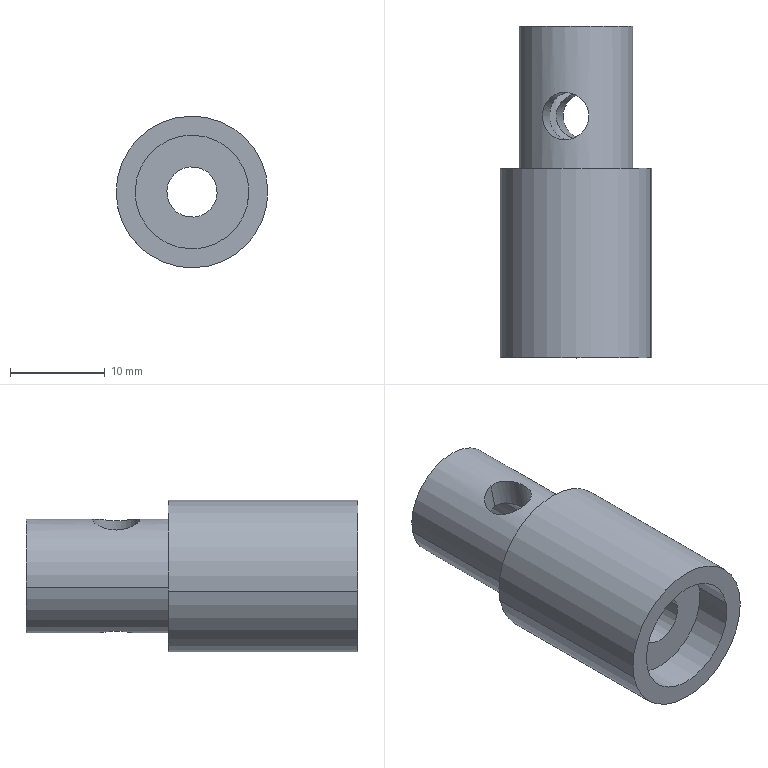Component | SolidWorks | UltrasonicProductSuction-10_SuctionPositioning-1 | 1 solid | 19 faces | box 16 x 35 x 16 mm | volume 4290 mm3 | cylinder 14 | plane 5 | commonest cylinder face diameters 5 x4 12 x4 5.3 x2 16 x2 6 x2 | material AISI 304
STEP:
#1=COLOUR_RGB('',0.7922,0.8196,0.9333);
#2=FILL_AREA_STYLE_COLOUR('',#1);
#3=FILL_AREA_STYLE('',(#2));
#4=SURFACE_STYLE_FILL_AREA(#3);
#5=SURFACE_SIDE_STYLE('',(#4));
#6=SURFACE_STYLE_USAGE(.BOTH.,#5);
#7=PRESENTATION_STYLE_ASSIGNMENT((#6));
#8=CARTESIAN_POINT('',(68.99,150.659,43.813));
#9=VERTEX_POINT('',#8);
#10=CARTESIAN_POINT('',(68.99,150.855,43.813));
#11=VERTEX_POINT('',#10);
#12=CARTESIAN_POINT('',(68.99,150.659,43.813));
#13=CARTESIAN_POINT('',(68.984,150.659,43.812));
#14=CARTESIAN_POINT('',(68.978,150.659,43.811));
#15=CARTESIAN_POINT('',(68.965,150.662,43.81));
#16=CARTESIAN_POINT('',(68.959,150.664,43.809));
#17=CARTESIAN_POINT('',(68.941,150.671,43.808));
#18=CARTESIAN_POINT('',(68.929,150.678,43.809));
#19=CARTESIAN_POINT('',(68.915,150.692,43.81));
#20=CARTESIAN_POINT('',(68.911,150.697,43.811));
#21=CARTESIAN_POINT('',(68.904,150.708,43.812));
#22=CARTESIAN_POINT('',(68.9,150.713,43.813));
#23=CARTESIAN_POINT('',(68.895,150.725,43.814));
#24=CARTESIAN_POINT('',(68.893,150.731,43.814));
#25=CARTESIAN_POINT('',(68.89,150.744,43.815));
#26=CARTESIAN_POINT('',(68.89,150.75,43.815));
#27=CARTESIAN_POINT('',(68.89,150.77,43.815));
#28=CARTESIAN_POINT('',(68.892,150.783,43.814));
#29=CARTESIAN_POINT('',(68.9,150.801,43.813));
#30=CARTESIAN_POINT('',(68.904,150.807,43.812));
#31=CARTESIAN_POINT('',(68.911,150.817,43.811));
#32=CARTESIAN_POINT('',(68.915,150.822,43.81));
#33=CARTESIAN_POINT('',(68.929,150.836,43.809));
#34=CARTESIAN_POINT('',(68.941,150.843,43.808));
#35=CARTESIAN_POINT('',(68.959,150.85,43.809));
#36=CARTESIAN_POINT('',(68.965,150.852,43.81));
#37=CARTESIAN_POINT('',(68.978,150.855,43.811));
#38=CARTESIAN_POINT('',(68.984,150.855,43.812));
#39=CARTESIAN_POINT('',(68.99,150.855,43.813));
#40=B_SPLINE_CURVE_WITH_KNOTS('',3,(#12,#13,#14,#15,#16,#17,#18,#19,#20,#21,#22,#23,#24,#25,#26,#27,#28,#29,#30,#31,#32,#33,#34,#35,#36,#37,#38,#39),.UNSPECIFIED.,.F.,.F.,(4,2,2,2,2,2,2,2,2,2,2,2,2,4),(0.00756,0.008054,0.008548,0.009536,0.01003,0.01052,0.01102,0.01151,0.0125,0.01299,0.01349,0.01447,0.01497,0.01546),.UNSPECIFIED.);
#41=EDGE_CURVE('',#9,#11,#40,.T.);
#42=ORIENTED_EDGE('',*,*,#41,.T.);
#43=CARTESIAN_POINT('',(68.967,150.855,43.929));
#44=VERTEX_POINT('',#43);
#45=CARTESIAN_POINT('',(69.006,150.855,43.736));
#46=DIRECTION('',(-0.1987,-0.00003085,0.9801));
#47=VECTOR('',#46,39.37);
#48=LINE('',#45,#47);
#49=EDGE_CURVE('',#11,#44,#48,.T.);
#50=ORIENTED_EDGE('',*,*,#49,.T.);
#51=CARTESIAN_POINT('',(68.967,150.659,43.929));
#52=VERTEX_POINT('',#51);
#53=CARTESIAN_POINT('',(68.967,150.659,43.929));
#54=CARTESIAN_POINT('',(68.96,150.659,43.928));
#55=CARTESIAN_POINT('',(68.953,150.659,43.927));
#56=CARTESIAN_POINT('',(68.94,150.662,43.927));
#57=CARTESIAN_POINT('',(68.933,150.664,43.927));
#58=CARTESIAN_POINT('',(68.921,150.669,43.929));
#59=CARTESIAN_POINT('',(68.915,150.673,43.93));
#60=CARTESIAN_POINT('',(68.903,150.68,43.934));
#61=CARTESIAN_POINT('',(68.898,150.684,43.936));
#62=CARTESIAN_POINT('',(68.889,150.693,43.94));
#63=CARTESIAN_POINT('',(68.884,150.697,43.943));
#64=CARTESIAN_POINT('',(68.876,150.707,43.948));
#65=CARTESIAN_POINT('',(68.873,150.713,43.95));
#66=CARTESIAN_POINT('',(68.867,150.724,43.955));
#67=CARTESIAN_POINT('',(68.864,150.73,43.957));
#68=CARTESIAN_POINT('',(68.862,150.74,43.96));
#69=CARTESIAN_POINT('',(68.861,150.743,43.96));
#70=CARTESIAN_POINT('',(68.86,150.75,43.961));
#71=CARTESIAN_POINT('',(68.86,150.754,43.961));
#72=CARTESIAN_POINT('',(68.86,150.764,43.961));
#73=CARTESIAN_POINT('',(68.861,150.771,43.96));
#74=CARTESIAN_POINT('',(68.864,150.784,43.957));
#75=CARTESIAN_POINT('',(68.867,150.79,43.955));
#76=CARTESIAN_POINT('',(68.873,150.801,43.95));
#77=CARTESIAN_POINT('',(68.876,150.807,43.948));
#78=CARTESIAN_POINT('',(68.884,150.817,43.943));
#79=CARTESIAN_POINT('',(68.889,150.821,43.94));
#80=CARTESIAN_POINT('',(68.898,150.83,43.936));
#81=CARTESIAN_POINT('',(68.903,150.834,43.934));
#82=CARTESIAN_POINT('',(68.915,150.841,43.93));
#83=CARTESIAN_POINT('',(68.92,150.844,43.929));
#84=CARTESIAN_POINT('',(68.933,150.85,43.927));
#85=CARTESIAN_POINT('',(68.94,150.852,43.927));
#86=CARTESIAN_POINT('',(68.953,150.855,43.927));
#87=CARTESIAN_POINT('',(68.96,150.855,43.928));
#88=CARTESIAN_POINT('',(68.967,150.855,43.929));
#89=B_SPLINE_CURVE_WITH_KNOTS('',3,(#53,#54,#55,#56,#57,#58,#59,#60,#61,#62,#63,#64,#65,#66,#67,#68,#69,#70,#71,#72,#73,#74,#75,#76,#77,#78,#79,#80,#81,#82,#83,#84,#85,#86,#87,#88),.UNSPECIFIED.,.F.,.F.,(4,2,2,2,2,2,2,2,2,2,2,2,2,2,2,2,2,4),(0.008234,0.008754,0.009273,0.009792,0.01031,0.01083,0.01135,0.01187,0.01213,0.01239,0.01291,0.01343,0.01395,0.01447,0.01499,0.01551,0.01602,0.01654),.UNSPECIFIED.);
#90=EDGE_CURVE('',#52,#44,#89,.T.);
#91=ORIENTED_EDGE('',*,*,#90,.F.);
#92=CARTESIAN_POINT('',(69.006,150.659,43.736));
#93=DIRECTION('',(-0.1987,-0.00003085,0.9801));
#94=VECTOR('',#93,39.37);
#95=LINE('',#92,#94);
#96=EDGE_CURVE('',#9,#52,#95,.T.);
#97=ORIENTED_EDGE('',*,*,#96,.F.);
#98=EDGE_LOOP('',(#42,#50,#91,#97));
#99=FACE_OUTER_BOUND('',#98,.T.);
#100=CARTESIAN_POINT('',(69.006,150.757,43.736));
#101=DIRECTION('',(-0.1987,-0.00003085,0.9801));
#102=DIRECTION('',(0.0001552,-1.,0.));
#103=AXIS2_PLACEMENT_3D('',#100,#101,#102);
#104=CYLINDRICAL_SURFACE('',#103,0.09843);
#105=ADVANCED_FACE('',(#99),#104,.F.);
#106=CARTESIAN_POINT('',(68.92,150.855,44.161));
#107=VERTEX_POINT('',#106);
#108=CARTESIAN_POINT('',(68.92,150.659,44.161));
#109=VERTEX_POINT('',#108);
#110=CARTESIAN_POINT('',(68.92,150.855,44.161));
#111=CARTESIAN_POINT('',(68.913,150.855,44.159));
#112=CARTESIAN_POINT('',(68.907,150.855,44.157));
#113=CARTESIAN_POINT('',(68.894,150.852,44.152));
#114=CARTESIAN_POINT('',(68.888,150.85,44.149));
#115=CARTESIAN_POINT('',(68.872,150.842,44.14));
#116=CARTESIAN_POINT('',(68.863,150.835,44.132));
#117=CARTESIAN_POINT('',(68.849,150.817,44.116));
#118=CARTESIAN_POINT('',(68.843,150.807,44.108));
#119=CARTESIAN_POINT('',(68.838,150.79,44.098));
#120=CARTESIAN_POINT('',(68.836,150.784,44.095));
#121=CARTESIAN_POINT('',(68.835,150.774,44.092));
#122=CARTESIAN_POINT('',(68.835,150.771,44.091));
#123=CARTESIAN_POINT('',(68.834,150.764,44.09));
#124=CARTESIAN_POINT('',(68.834,150.761,44.089));
#125=CARTESIAN_POINT('',(68.834,150.75,44.089));
#126=CARTESIAN_POINT('',(68.835,150.743,44.091));
#127=CARTESIAN_POINT('',(68.836,150.73,44.095));
#128=CARTESIAN_POINT('',(68.838,150.724,44.098));
#129=CARTESIAN_POINT('',(68.843,150.707,44.108));
#130=CARTESIAN_POINT('',(68.848,150.697,44.116));
#131=CARTESIAN_POINT('',(68.863,150.679,44.132));
#132=CARTESIAN_POINT('',(68.872,150.672,44.14));
#133=CARTESIAN_POINT('',(68.888,150.664,44.149));
#134=CARTESIAN_POINT('',(68.894,150.662,44.152));
#135=CARTESIAN_POINT('',(68.907,150.659,44.157));
#136=CARTESIAN_POINT('',(68.913,150.659,44.159));
#137=CARTESIAN_POINT('',(68.92,150.659,44.161));
#138=B_SPLINE_CURVE_WITH_KNOTS('',3,(#110,#111,#112,#113,#114,#115,#116,#117,#118,#119,#120,#121,#122,#123,#124,#125,#126,#127,#128,#129,#130,#131,#132,#133,#134,#135,#136,#137),.UNSPECIFIED.,.F.,.F.,(4,2,2,2,2,2,2,2,2,2,2,2,2,4),(0.01654,0.01707,0.01759,0.01863,0.01967,0.02019,0.02045,0.02071,0.02123,0.02175,0.0228,0.02384,0.02436,0.02488),.UNSPECIFIED.);
#139=EDGE_CURVE('',#107,#109,#138,.T.);
#140=ORIENTED_EDGE('',*,*,#139,.F.);
#141=CARTESIAN_POINT('',(68.897,150.855,44.276));
#142=VERTEX_POINT('',#141);
#143=CARTESIAN_POINT('',(69.006,150.855,43.736));
#144=DIRECTION('',(-0.1987,-0.00003085,0.9801));
#145=VECTOR('',#144,39.37);
#146=LINE('',#143,#145);
#147=EDGE_CURVE('',#107,#142,#146,.T.);
#148=ORIENTED_EDGE('',*,*,#147,.T.);
#149=CARTESIAN_POINT('',(68.897,150.659,44.276));
#150=VERTEX_POINT('',#149);
#151=CARTESIAN_POINT('',(68.897,150.855,44.276));
#152=CARTESIAN_POINT('',(68.89,150.855,44.275));
#153=CARTESIAN_POINT('',(68.884,150.855,44.274));
#154=CARTESIAN_POINT('',(68.871,150.852,44.27));
#155=CARTESIAN_POINT('',(68.866,150.85,44.268));
#156=CARTESIAN_POINT('',(68.854,150.845,44.264));
#157=CARTESIAN_POINT('',(68.849,150.842,44.261));
#158=CARTESIAN_POINT('',(68.839,150.835,44.257));
#159=CARTESIAN_POINT('',(68.834,150.831,44.255));
#160=CARTESIAN_POINT('',(68.826,150.822,44.25));
#161=CARTESIAN_POINT('',(68.822,150.817,44.248));
#162=CARTESIAN_POINT('',(68.816,150.806,44.244));
#163=CARTESIAN_POINT('',(68.813,150.801,44.242));
#164=CARTESIAN_POINT('',(68.809,150.789,44.239));
#165=CARTESIAN_POINT('',(68.807,150.783,44.238));
#166=CARTESIAN_POINT('',(68.805,150.77,44.236));
#167=CARTESIAN_POINT('',(68.804,150.763,44.236));
#168=CARTESIAN_POINT('',(68.804,150.75,44.236));
#169=CARTESIAN_POINT('',(68.805,150.744,44.236));
#170=CARTESIAN_POINT('',(68.807,150.731,44.238));
#171=CARTESIAN_POINT('',(68.809,150.725,44.239));
#172=CARTESIAN_POINT('',(68.813,150.713,44.242));
#173=CARTESIAN_POINT('',(68.816,150.707,44.244));
#174=CARTESIAN_POINT('',(68.823,150.697,44.248));
#175=CARTESIAN_POINT('',(68.826,150.692,44.25));
#176=CARTESIAN_POINT('',(68.835,150.683,44.255));
#177=CARTESIAN_POINT('',(68.839,150.679,44.257));
#178=CARTESIAN_POINT('',(68.849,150.672,44.262));
#179=CARTESIAN_POINT('',(68.854,150.669,44.264));
#180=CARTESIAN_POINT('',(68.871,150.661,44.27));
#181=CARTESIAN_POINT('',(68.884,150.659,44.274));
#182=CARTESIAN_POINT('',(68.897,150.659,44.276));
#183=B_SPLINE_CURVE_WITH_KNOTS('',3,(#151,#152,#153,#154,#155,#156,#157,#158,#159,#160,#161,#162,#163,#164,#165,#166,#167,#168,#169,#170,#171,#172,#173,#174,#175,#176,#177,#178,#179,#180,#181,#182),.UNSPECIFIED.,.F.,.F.,(4,2,2,2,2,2,2,2,2,2,2,2,2,2,2,4),(0.01546,0.01596,0.01645,0.01694,0.01744,0.01793,0.01843,0.01892,0.01941,0.01991,0.0204,0.0209,0.02139,0.02188,0.02238,0.02337),.UNSPECIFIED.);
#184=EDGE_CURVE('',#142,#150,#183,.T.);
#185=ORIENTED_EDGE('',*,*,#184,.T.);
#186=CARTESIAN_POINT('',(69.006,150.659,43.736));
#187=DIRECTION('',(-0.1987,-0.00003085,0.9801));
#188=VECTOR('',#187,39.37);
#189=LINE('',#186,#188);
#190=EDGE_CURVE('',#109,#150,#189,.T.);
#191=ORIENTED_EDGE('',*,*,#190,.F.);
#192=EDGE_LOOP('',(#140,#148,#185,#191));
#193=FACE_OUTER_BOUND('',#192,.T.);
#194=CARTESIAN_POINT('',(69.006,150.757,43.736));
#195=DIRECTION('',(-0.1987,-0.00003085,0.9801));
#196=DIRECTION('',(0.0001552,-1.,0.));
#197=AXIS2_PLACEMENT_3D('',#194,#195,#196);
#198=CYLINDRICAL_SURFACE('',#197,0.09843);
#199=ADVANCED_FACE('',(#193),#198,.F.);
#200=CARTESIAN_POINT('',(68.841,149.911,44.024));
#201=VERTEX_POINT('',#200);
#202=CARTESIAN_POINT('',(69.046,149.911,44.066));
#203=VERTEX_POINT('',#202);
#204=CARTESIAN_POINT('',(68.944,149.911,44.045));
#205=DIRECTION('',(0.0001552,-1.,0.));
#206=DIRECTION('',(0.9801,0.0001522,0.1987));
#207=AXIS2_PLACEMENT_3D('',#204,#205,#206);
#208=CIRCLE('',#207,0.1043);
#209=EDGE_CURVE('',#201,#203,#208,.T.);
#210=ORIENTED_EDGE('',*,*,#209,.T.);
#211=CARTESIAN_POINT('',(69.046,150.068,44.066));
#212=VERTEX_POINT('',#211);
#213=CARTESIAN_POINT('',(69.046,149.871,44.066));
#214=DIRECTION('',(-0.0001552,1.,-0.));
#215=VECTOR('',#214,39.37);
#216=LINE('',#213,#215);
#217=EDGE_CURVE('',#203,#212,#216,.T.);
#218=ORIENTED_EDGE('',*,*,#217,.T.);
#219=CARTESIAN_POINT('',(68.841,150.068,44.024));
#220=VERTEX_POINT('',#219);
#221=CARTESIAN_POINT('',(68.944,150.068,44.045));
#222=DIRECTION('',(-0.0001552,1.,-0.));
#223=DIRECTION('',(-0.9801,-0.0001522,-0.1987));
#224=AXIS2_PLACEMENT_3D('',#221,#222,#223);
#225=CIRCLE('',#224,0.1043);
#226=EDGE_CURVE('',#212,#220,#225,.T.);
#227=ORIENTED_EDGE('',*,*,#226,.T.);
#228=CARTESIAN_POINT('',(68.841,149.871,44.024));
#229=DIRECTION('',(-0.0001552,1.,-0.));
#230=VECTOR('',#229,39.37);
#231=LINE('',#228,#230);
#232=EDGE_CURVE('',#201,#220,#231,.T.);
#233=ORIENTED_EDGE('',*,*,#232,.F.);
#234=EDGE_LOOP('',(#210,#218,#227,#233));
#235=FACE_OUTER_BOUND('',#234,.T.);
#236=CARTESIAN_POINT('',(68.944,149.871,44.045));
#237=DIRECTION('',(-0.0001552,1.,-0.));
#238=DIRECTION('',(-0.9801,-0.0001522,-0.1987));
#239=AXIS2_PLACEMENT_3D('',#236,#237,#238);
#240=CYLINDRICAL_SURFACE('',#239,0.1043);
#241=ADVANCED_FACE('',(#235),#240,.F.);
#242=CARTESIAN_POINT('',(68.712,149.911,43.998));
#243=VERTEX_POINT('',#242);
#244=CARTESIAN_POINT('',(69.175,149.911,44.092));
#245=VERTEX_POINT('',#244);
#246=CARTESIAN_POINT('',(68.944,149.911,44.045));
#247=DIRECTION('',(0.0001552,-1.,0.));
#248=DIRECTION('',(0.9801,0.0001522,0.1987));
#249=AXIS2_PLACEMENT_3D('',#246,#247,#248);
#250=CIRCLE('',#249,0.2362);
#251=EDGE_CURVE('',#243,#245,#250,.T.);
#252=ORIENTED_EDGE('',*,*,#251,.F.);
#253=CARTESIAN_POINT('',(68.712,149.753,43.998));
#254=VERTEX_POINT('',#253);
#255=CARTESIAN_POINT('',(68.712,149.911,43.998));
#256=DIRECTION('',(0.0001552,-1.,0.));
#257=VECTOR('',#256,39.37);
#258=LINE('',#255,#257);
#259=EDGE_CURVE('',#243,#254,#258,.T.);
#260=ORIENTED_EDGE('',*,*,#259,.T.);
#261=CARTESIAN_POINT('',(69.175,149.753,44.092));
#262=VERTEX_POINT('',#261);
#263=CARTESIAN_POINT('',(68.944,149.753,44.045));
#264=DIRECTION('',(0.0001552,-1.,0.));
#265=DIRECTION('',(0.9801,0.0001522,0.1987));
#266=AXIS2_PLACEMENT_3D('',#263,#264,#265);
#267=CIRCLE('',#266,0.2362);
#268=EDGE_CURVE('',#254,#262,#267,.T.);
#269=ORIENTED_EDGE('',*,*,#268,.T.);
#270=CARTESIAN_POINT('',(69.175,149.911,44.092));
#271=DIRECTION('',(0.0001552,-1.,0.));
#272=VECTOR('',#271,39.37);
#273=LINE('',#270,#272);
#274=EDGE_CURVE('',#245,#262,#273,.T.);
#275=ORIENTED_EDGE('',*,*,#274,.F.);
#276=EDGE_LOOP('',(#252,#260,#269,#275));
#277=FACE_OUTER_BOUND('',#276,.T.);
#278=CARTESIAN_POINT('',(68.944,149.911,44.045));
#279=DIRECTION('',(0.0001552,-1.,0.));
#280=DIRECTION('',(0.9801,0.0001522,0.1987));
#281=AXIS2_PLACEMENT_3D('',#278,#279,#280);
#282=CYLINDRICAL_SURFACE('',#281,0.2362);
#283=ADVANCED_FACE('',(#277),#282,.F.);
#284=CARTESIAN_POINT('',(69.252,149.753,44.108));
#285=VERTEX_POINT('',#284);
#286=CARTESIAN_POINT('',(68.635,149.753,43.982));
#287=VERTEX_POINT('',#286);
#288=CARTESIAN_POINT('',(68.944,149.753,44.045));
#289=DIRECTION('',(0.0001552,-1.,0.));
#290=DIRECTION('',(0.9801,0.0001522,0.1987));
#291=AXIS2_PLACEMENT_3D('',#288,#289,#290);
#292=CIRCLE('',#291,0.315);
#293=EDGE_CURVE('',#285,#287,#292,.T.);
#294=ORIENTED_EDGE('',*,*,#293,.F.);
#295=CARTESIAN_POINT('',(69.252,150.541,44.108));
#296=VERTEX_POINT('',#295);
#297=CARTESIAN_POINT('',(69.252,149.556,44.108));
#298=DIRECTION('',(-0.0001552,1.,-0.));
#299=VECTOR('',#298,39.37);
#300=LINE('',#297,#299);
#301=EDGE_CURVE('',#285,#296,#300,.T.);
#302=ORIENTED_EDGE('',*,*,#301,.T.);
#303=CARTESIAN_POINT('',(68.635,150.54,43.982));
#304=VERTEX_POINT('',#303);
#305=CARTESIAN_POINT('',(68.943,150.54,44.045));
#306=DIRECTION('',(-0.0001552,1.,-0.));
#307=DIRECTION('',(-0.9801,-0.0001522,-0.1987));
#308=AXIS2_PLACEMENT_3D('',#305,#306,#307);
#309=CIRCLE('',#308,0.315);
#310=EDGE_CURVE('',#304,#296,#309,.T.);
#311=ORIENTED_EDGE('',*,*,#310,.F.);
#312=CARTESIAN_POINT('',(68.635,149.556,43.982));
#313=DIRECTION('',(-0.0001552,1.,-0.));
#314=VECTOR('',#313,39.37);
#315=LINE('',#312,#314);
#316=EDGE_CURVE('',#287,#304,#315,.T.);
#317=ORIENTED_EDGE('',*,*,#316,.F.);
#318=EDGE_LOOP('',(#294,#302,#311,#317));
#319=FACE_OUTER_BOUND('',#318,.T.);
#320=CARTESIAN_POINT('',(68.944,149.556,44.045));
#321=DIRECTION('',(-0.0001552,1.,-0.));
#322=DIRECTION('',(-0.9801,-0.0001522,-0.1987));
#323=AXIS2_PLACEMENT_3D('',#320,#321,#322);
#324=CYLINDRICAL_SURFACE('',#323,0.315);
#325=ADVANCED_FACE('',(#319),#324,.T.);
#326=CARTESIAN_POINT('',(68.897,150.659,44.276));
#327=CARTESIAN_POINT('',(68.903,150.659,44.278));
#328=CARTESIAN_POINT('',(68.909,150.659,44.279));
#329=CARTESIAN_POINT('',(68.922,150.662,44.28));
#330=CARTESIAN_POINT('',(68.928,150.664,44.281));
#331=CARTESIAN_POINT('',(68.946,150.671,44.281));
#332=CARTESIAN_POINT('',(68.958,150.678,44.281));
#333=CARTESIAN_POINT('',(68.972,150.692,44.28));
#334=CARTESIAN_POINT('',(68.976,150.697,44.279));
#335=CARTESIAN_POINT('',(68.983,150.708,44.278));
#336=CARTESIAN_POINT('',(68.987,150.713,44.277));
#337=CARTESIAN_POINT('',(68.992,150.725,44.276));
#338=CARTESIAN_POINT('',(68.994,150.731,44.276));
#339=CARTESIAN_POINT('',(68.997,150.744,44.275));
#340=CARTESIAN_POINT('',(68.997,150.75,44.275));
#341=CARTESIAN_POINT('',(68.997,150.77,44.275));
#342=CARTESIAN_POINT('',(68.994,150.783,44.276));
#343=CARTESIAN_POINT('',(68.986,150.801,44.277));
#344=CARTESIAN_POINT('',(68.983,150.807,44.278));
#345=CARTESIAN_POINT('',(68.976,150.817,44.279));
#346=CARTESIAN_POINT('',(68.971,150.822,44.28));
#347=CARTESIAN_POINT('',(68.957,150.836,44.281));
#348=CARTESIAN_POINT('',(68.946,150.843,44.281));
#349=CARTESIAN_POINT('',(68.928,150.85,44.281));
#350=CARTESIAN_POINT('',(68.922,150.852,44.28));
#351=CARTESIAN_POINT('',(68.909,150.855,44.279));
#352=CARTESIAN_POINT('',(68.903,150.855,44.278));
#353=CARTESIAN_POINT('',(68.897,150.855,44.276));
#354=B_SPLINE_CURVE_WITH_KNOTS('',3,(#326,#327,#328,#329,#330,#331,#332,#333,#334,#335,#336,#337,#338,#339,#340,#341,#342,#343,#344,#345,#346,#347,#348,#349,#350,#351,#352,#353),.UNSPECIFIED.,.F.,.F.,(4,2,2,2,2,2,2,2,2,2,2,2,2,4),(0.00756,0.008054,0.008548,0.009536,0.01003,0.01052,0.01102,0.01151,0.0125,0.01299,0.01349,0.01447,0.01497,0.01546),.UNSPECIFIED.);
#355=EDGE_CURVE('',#150,#142,#354,.T.);
#356=ORIENTED_EDGE('',*,*,#355,.F.);
#357=ORIENTED_EDGE('',*,*,#184,.F.);
#358=EDGE_LOOP('',(#356,#357));
#359=FACE_BOUND('',#358,.T.);
#360=CARTESIAN_POINT('',(68.712,150.54,43.998));
#361=VERTEX_POINT('',#360);
#362=CARTESIAN_POINT('',(69.175,150.541,44.092));
#363=VERTEX_POINT('',#362);
#364=CARTESIAN_POINT('',(68.943,150.54,44.045));
#365=DIRECTION('',(-0.0001552,1.,-0.));
#366=DIRECTION('',(-0.9801,-0.0001522,-0.1987));
#367=AXIS2_PLACEMENT_3D('',#364,#365,#366);
#368=CIRCLE('',#367,0.2362);
#369=EDGE_CURVE('',#361,#363,#368,.T.);
#370=ORIENTED_EDGE('',*,*,#369,.T.);
#371=CARTESIAN_POINT('',(69.175,151.131,44.092));
#372=VERTEX_POINT('',#371);
#373=CARTESIAN_POINT('',(69.175,150.147,44.092));
#374=DIRECTION('',(-0.0001552,1.,-0.));
#375=VECTOR('',#374,39.37);
#376=LINE('',#373,#375);
#377=EDGE_CURVE('',#363,#372,#376,.T.);
#378=ORIENTED_EDGE('',*,*,#377,.T.);
#379=CARTESIAN_POINT('',(68.712,151.131,43.998));
#380=VERTEX_POINT('',#379);
#381=CARTESIAN_POINT('',(68.943,151.131,44.045));
#382=DIRECTION('',(-0.0001552,1.,-0.));
#383=DIRECTION('',(-0.9801,-0.0001522,-0.1987));
#384=AXIS2_PLACEMENT_3D('',#381,#382,#383);
#385=CIRCLE('',#384,0.2362);
#386=EDGE_CURVE('',#380,#372,#385,.T.);
#387=ORIENTED_EDGE('',*,*,#386,.F.);
#388=CARTESIAN_POINT('',(68.712,150.147,43.998));
#389=DIRECTION('',(-0.0001552,1.,-0.));
#390=VECTOR('',#389,39.37);
#391=LINE('',#388,#390);
#392=EDGE_CURVE('',#361,#380,#391,.T.);
#393=ORIENTED_EDGE('',*,*,#392,.F.);
#394=EDGE_LOOP('',(#370,#378,#387,#393));
#395=FACE_OUTER_BOUND('',#394,.T.);
#396=CARTESIAN_POINT('',(68.944,150.147,44.045));
#397=DIRECTION('',(-0.0001552,1.,-0.));
#398=DIRECTION('',(-0.9801,-0.0001522,-0.1987));
#399=AXIS2_PLACEMENT_3D('',#396,#397,#398);
#400=CYLINDRICAL_SURFACE('',#399,0.2362);
#401=ADVANCED_FACE('',(#359,#395),#400,.T.);
#402=ORIENTED_EDGE('',*,*,#90,.T.);
#403=CARTESIAN_POINT('',(68.967,150.855,43.929));
#404=CARTESIAN_POINT('',(68.974,150.855,43.931));
#405=CARTESIAN_POINT('',(68.98,150.855,43.933));
#406=CARTESIAN_POINT('',(68.993,150.852,43.937));
#407=CARTESIAN_POINT('',(68.999,150.85,43.94));
#408=CARTESIAN_POINT('',(69.015,150.842,43.95));
#409=CARTESIAN_POINT('',(69.024,150.835,43.958));
#410=CARTESIAN_POINT('',(69.038,150.817,43.974));
#411=CARTESIAN_POINT('',(69.044,150.807,43.982));
#412=CARTESIAN_POINT('',(69.049,150.79,43.992));
#413=CARTESIAN_POINT('',(69.05,150.784,43.995));
#414=CARTESIAN_POINT('',(69.052,150.774,43.998));
#415=CARTESIAN_POINT('',(69.052,150.771,43.999));
#416=CARTESIAN_POINT('',(69.053,150.764,44.));
#417=CARTESIAN_POINT('',(69.053,150.761,44.));
#418=CARTESIAN_POINT('',(69.053,150.75,44.001));
#419=CARTESIAN_POINT('',(69.052,150.743,43.999));
#420=CARTESIAN_POINT('',(69.051,150.73,43.995));
#421=CARTESIAN_POINT('',(69.049,150.724,43.992));
#422=CARTESIAN_POINT('',(69.044,150.707,43.982));
#423=CARTESIAN_POINT('',(69.038,150.697,43.974));
#424=CARTESIAN_POINT('',(69.024,150.679,43.958));
#425=CARTESIAN_POINT('',(69.015,150.672,43.95));
#426=CARTESIAN_POINT('',(68.999,150.664,43.94));
#427=CARTESIAN_POINT('',(68.993,150.662,43.937));
#428=CARTESIAN_POINT('',(68.98,150.659,43.933));
#429=CARTESIAN_POINT('',(68.974,150.659,43.931));
#430=CARTESIAN_POINT('',(68.967,150.659,43.929));
#431=B_SPLINE_CURVE_WITH_KNOTS('',3,(#403,#404,#405,#406,#407,#408,#409,#410,#411,#412,#413,#414,#415,#416,#417,#418,#419,#420,#421,#422,#423,#424,#425,#426,#427,#428,#429,#430),.UNSPECIFIED.,.F.,.F.,(4,2,2,2,2,2,2,2,2,2,2,2,2,4),(0.01654,0.01707,0.01759,0.01863,0.01967,0.02019,0.02045,0.02071,0.02123,0.02175,0.0228,0.02384,0.02436,0.02488),.UNSPECIFIED.);
#432=EDGE_CURVE('',#44,#52,#431,.T.);
#433=ORIENTED_EDGE('',*,*,#432,.T.);
#434=EDGE_LOOP('',(#402,#433));
#435=FACE_BOUND('',#434,.T.);
#436=CARTESIAN_POINT('',(69.059,150.068,44.068));
#437=VERTEX_POINT('',#436);
#438=CARTESIAN_POINT('',(68.828,150.068,44.021));
#439=VERTEX_POINT('',#438);
#440=CARTESIAN_POINT('',(68.944,150.068,44.045));
#441=DIRECTION('',(-0.0001552,1.,-0.));
#442=DIRECTION('',(-0.9801,-0.0001522,-0.1987));
#443=AXIS2_PLACEMENT_3D('',#440,#441,#442);
#444=CIRCLE('',#443,0.1181);
#445=EDGE_CURVE('',#437,#439,#444,.T.);
#446=ORIENTED_EDGE('',*,*,#445,.F.);
#447=CARTESIAN_POINT('',(69.059,151.131,44.068));
#448=VERTEX_POINT('',#447);
#449=CARTESIAN_POINT('',(69.059,150.068,44.068));
#450=DIRECTION('',(-0.0001552,1.,-0.));
#451=VECTOR('',#450,39.37);
#452=LINE('',#449,#451);
#453=EDGE_CURVE('',#437,#448,#452,.T.);
#454=ORIENTED_EDGE('',*,*,#453,.T.);
#455=CARTESIAN_POINT('',(68.828,151.131,44.021));
#456=VERTEX_POINT('',#455);
#457=CARTESIAN_POINT('',(68.943,151.131,44.045));
#458=DIRECTION('',(-0.0001552,1.,-0.));
#459=DIRECTION('',(-0.9801,-0.0001522,-0.1987));
#460=AXIS2_PLACEMENT_3D('',#457,#458,#459);
#461=CIRCLE('',#460,0.1181);
#462=EDGE_CURVE('',#448,#456,#461,.T.);
#463=ORIENTED_EDGE('',*,*,#462,.T.);
#464=CARTESIAN_POINT('',(68.828,150.068,44.021));
#465=DIRECTION('',(-0.0001552,1.,-0.));
#466=VECTOR('',#465,39.37);
#467=LINE('',#464,#466);
#468=EDGE_CURVE('',#439,#456,#467,.T.);
#469=ORIENTED_EDGE('',*,*,#468,.F.);
#470=EDGE_LOOP('',(#446,#454,#463,#469));
#471=FACE_OUTER_BOUND('',#470,.T.);
#472=CARTESIAN_POINT('',(68.944,150.068,44.045));
#473=DIRECTION('',(-0.0001552,1.,-0.));
#474=DIRECTION('',(-0.9801,-0.0001522,-0.1987));
#475=AXIS2_PLACEMENT_3D('',#472,#473,#474);
#476=CYLINDRICAL_SURFACE('',#475,0.1181);
#477=ADVANCED_FACE('',(#435,#471),#476,.F.);
#478=CARTESIAN_POINT('',(68.943,151.131,44.045));
#479=DIRECTION('',(-0.0001552,1.,-0.));
#480=DIRECTION('',(-0.9801,-0.0001522,-0.1987));
#481=AXIS2_PLACEMENT_3D('',#478,#479,#480);
#482=CIRCLE('',#481,0.1181);
#483=EDGE_CURVE('',#456,#448,#482,.T.);
#484=ORIENTED_EDGE('',*,*,#483,.F.);
#485=ORIENTED_EDGE('',*,*,#462,.F.);
#486=EDGE_LOOP('',(#484,#485));
#487=FACE_BOUND('',#486,.T.);
#488=ORIENTED_EDGE('',*,*,#386,.T.);
#489=CARTESIAN_POINT('',(68.943,151.131,44.045));
#490=DIRECTION('',(-0.0001552,1.,-0.));
#491=DIRECTION('',(-0.9801,-0.0001522,-0.1987));
#492=AXIS2_PLACEMENT_3D('',#489,#490,#491);
#493=CIRCLE('',#492,0.2362);
#494=EDGE_CURVE('',#372,#380,#493,.T.);
#495=ORIENTED_EDGE('',*,*,#494,.T.);
#496=EDGE_LOOP('',(#488,#495));
#497=FACE_OUTER_BOUND('',#496,.T.);
#498=CARTESIAN_POINT('',(68.943,151.131,44.045));
#499=DIRECTION('',(0.0001552,-1.,0.));
#500=DIRECTION('',(0.9801,0.0001522,0.1987));
#501=AXIS2_PLACEMENT_3D('',#498,#499,#500);
#502=PLANE('',#501);
#503=ADVANCED_FACE('',(#487,#497),#502,.F.);
#504=ORIENTED_EDGE('',*,*,#453,.F.);
#505=CARTESIAN_POINT('',(68.944,150.068,44.045));
#506=DIRECTION('',(-0.0001552,1.,-0.));
#507=DIRECTION('',(-0.9801,-0.0001522,-0.1987));
#508=AXIS2_PLACEMENT_3D('',#505,#506,#507);
#509=CIRCLE('',#508,0.1181);
#510=EDGE_CURVE('',#439,#437,#509,.T.);
#511=ORIENTED_EDGE('',*,*,#510,.F.);
#512=ORIENTED_EDGE('',*,*,#468,.T.);
#513=ORIENTED_EDGE('',*,*,#483,.T.);
#514=EDGE_LOOP('',(#504,#511,#512,#513));
#515=FACE_OUTER_BOUND('',#514,.T.);
#516=CARTESIAN_POINT('',(68.92,150.659,44.161));
#517=CARTESIAN_POINT('',(68.927,150.659,44.162));
#518=CARTESIAN_POINT('',(68.934,150.659,44.163));
#519=CARTESIAN_POINT('',(68.947,150.662,44.163));
#520=CARTESIAN_POINT('',(68.954,150.664,44.163));
#521=CARTESIAN_POINT('',(68.966,150.669,44.161));
#522=CARTESIAN_POINT('',(68.972,150.673,44.16));
#523=CARTESIAN_POINT('',(68.984,150.68,44.156));
#524=CARTESIAN_POINT('',(68.989,150.684,44.154));
#525=CARTESIAN_POINT('',(68.998,150.693,44.15));
#526=CARTESIAN_POINT('',(69.003,150.697,44.147));
#527=CARTESIAN_POINT('',(69.011,150.707,44.142));
#528=CARTESIAN_POINT('',(69.014,150.713,44.14));
#529=CARTESIAN_POINT('',(69.02,150.724,44.135));
#530=CARTESIAN_POINT('',(69.023,150.73,44.133));
#531=CARTESIAN_POINT('',(69.025,150.74,44.13));
#532=CARTESIAN_POINT('',(69.026,150.743,44.13));
#533=CARTESIAN_POINT('',(69.027,150.75,44.129));
#534=CARTESIAN_POINT('',(69.027,150.754,44.128));
#535=CARTESIAN_POINT('',(69.027,150.764,44.128));
#536=CARTESIAN_POINT('',(69.026,150.771,44.129));
#537=CARTESIAN_POINT('',(69.023,150.784,44.133));
#538=CARTESIAN_POINT('',(69.02,150.79,44.135));
#539=CARTESIAN_POINT('',(69.014,150.801,44.14));
#540=CARTESIAN_POINT('',(69.011,150.807,44.142));
#541=CARTESIAN_POINT('',(69.003,150.817,44.147));
#542=CARTESIAN_POINT('',(68.998,150.822,44.15));
#543=CARTESIAN_POINT('',(68.989,150.83,44.154));
#544=CARTESIAN_POINT('',(68.983,150.834,44.156));
#545=CARTESIAN_POINT('',(68.972,150.841,44.16));
#546=CARTESIAN_POINT('',(68.966,150.845,44.161));
#547=CARTESIAN_POINT('',(68.954,150.85,44.163));
#548=CARTESIAN_POINT('',(68.947,150.852,44.163));
#549=CARTESIAN_POINT('',(68.934,150.855,44.163));
#550=CARTESIAN_POINT('',(68.927,150.855,44.162));
#551=CARTESIAN_POINT('',(68.92,150.855,44.161));
#552=B_SPLINE_CURVE_WITH_KNOTS('',3,(#516,#517,#518,#519,#520,#521,#522,#523,#524,#525,#526,#527,#528,#529,#530,#531,#532,#533,#534,#535,#536,#537,#538,#539,#540,#541,#542,#543,#544,#545,#546,#547,#548,#549,#550,#551),.UNSPECIFIED.,.F.,.F.,(4,2,2,2,2,2,2,2,2,2,2,2,2,2,2,2,2,4),(0.008234,0.008754,0.009273,0.009792,0.01031,0.01083,0.01135,0.01187,0.01213,0.01239,0.01291,0.01343,0.01395,0.01447,0.01499,0.01551,0.01602,0.01654),.UNSPECIFIED.);
#553=EDGE_CURVE('',#109,#107,#552,.T.);
#554=ORIENTED_EDGE('',*,*,#553,.T.);
#555=ORIENTED_EDGE('',*,*,#139,.T.);
#556=EDGE_LOOP('',(#554,#555));
#557=FACE_BOUND('',#556,.T.);
#558=CARTESIAN_POINT('',(68.944,150.068,44.045));
#559=DIRECTION('',(-0.0001552,1.,-0.));
#560=DIRECTION('',(-0.9801,-0.0001522,-0.1987));
#561=AXIS2_PLACEMENT_3D('',#558,#559,#560);
#562=CYLINDRICAL_SURFACE('',#561,0.1181);
#563=ADVANCED_FACE('',(#515,#557),#562,.F.);
#564=CARTESIAN_POINT('',(68.944,150.068,44.045));
#565=DIRECTION('',(-0.0001552,1.,-0.));
#566=DIRECTION('',(-0.9801,-0.0001522,-0.1987));
#567=AXIS2_PLACEMENT_3D('',#564,#565,#566);
#568=CIRCLE('',#567,0.1043);
#569=EDGE_CURVE('',#220,#212,#568,.T.);
#570=ORIENTED_EDGE('',*,*,#569,.F.);
#571=ORIENTED_EDGE('',*,*,#226,.F.);
#572=EDGE_LOOP('',(#570,#571));
#573=FACE_BOUND('',#572,.T.);
#574=ORIENTED_EDGE('',*,*,#510,.T.);
#575=ORIENTED_EDGE('',*,*,#445,.T.);
#576=EDGE_LOOP('',(#574,#575));
#577=FACE_OUTER_BOUND('',#576,.T.);
#578=CARTESIAN_POINT('',(68.944,150.068,44.045));
#579=DIRECTION('',(-0.0001552,1.,-0.));
#580=DIRECTION('',(-0.9801,-0.0001522,-0.1987));
#581=AXIS2_PLACEMENT_3D('',#578,#579,#580);
#582=PLANE('',#581);
#583=ADVANCED_FACE('',(#573,#577),#582,.T.);
#584=ORIENTED_EDGE('',*,*,#369,.F.);
#585=CARTESIAN_POINT('',(68.943,150.54,44.045));
#586=DIRECTION('',(-0.0001552,1.,-0.));
#587=DIRECTION('',(-0.9801,-0.0001522,-0.1987));
#588=AXIS2_PLACEMENT_3D('',#585,#586,#587);
#589=CIRCLE('',#588,0.2362);
#590=EDGE_CURVE('',#363,#361,#589,.T.);
#591=ORIENTED_EDGE('',*,*,#590,.F.);
#592=EDGE_LOOP('',(#584,#591));
#593=FACE_BOUND('',#592,.T.);
#594=ORIENTED_EDGE('',*,*,#310,.T.);
#595=CARTESIAN_POINT('',(68.943,150.54,44.045));
#596=DIRECTION('',(-0.0001552,1.,-0.));
#597=DIRECTION('',(-0.9801,-0.0001522,-0.1987));
#598=AXIS2_PLACEMENT_3D('',#595,#596,#597);
#599=CIRCLE('',#598,0.315);
#600=EDGE_CURVE('',#296,#304,#599,.T.);
#601=ORIENTED_EDGE('',*,*,#600,.T.);
#602=EDGE_LOOP('',(#594,#601));
#603=FACE_OUTER_BOUND('',#602,.T.);
#604=CARTESIAN_POINT('',(68.943,150.54,44.045));
#605=DIRECTION('',(-0.0001552,1.,-0.));
#606=DIRECTION('',(-0.9801,-0.0001522,-0.1987));
#607=AXIS2_PLACEMENT_3D('',#604,#605,#606);
#608=PLANE('',#607);
#609=ADVANCED_FACE('',(#593,#603),#608,.T.);
#610=ORIENTED_EDGE('',*,*,#377,.F.);
#611=ORIENTED_EDGE('',*,*,#590,.T.);
#612=ORIENTED_EDGE('',*,*,#392,.T.);
#613=ORIENTED_EDGE('',*,*,#494,.F.);
#614=EDGE_LOOP('',(#610,#611,#612,#613));
#615=FACE_OUTER_BOUND('',#614,.T.);
#616=ORIENTED_EDGE('',*,*,#41,.F.);
#617=CARTESIAN_POINT('',(68.99,150.855,43.813));
#618=CARTESIAN_POINT('',(68.997,150.855,43.815));
#619=CARTESIAN_POINT('',(69.003,150.855,43.816));
#620=CARTESIAN_POINT('',(69.015,150.852,43.82));
#621=CARTESIAN_POINT('',(69.021,150.85,43.822));
#622=CARTESIAN_POINT('',(69.033,150.845,43.826));
#623=CARTESIAN_POINT('',(69.038,150.842,43.828));
#624=CARTESIAN_POINT('',(69.048,150.835,43.833));
#625=CARTESIAN_POINT('',(69.052,150.831,43.835));
#626=CARTESIAN_POINT('',(69.061,150.822,43.84));
#627=CARTESIAN_POINT('',(69.064,150.817,43.842));
#628=CARTESIAN_POINT('',(69.071,150.807,43.846));
#629=CARTESIAN_POINT('',(69.074,150.801,43.848));
#630=CARTESIAN_POINT('',(69.078,150.789,43.851));
#631=CARTESIAN_POINT('',(69.08,150.783,43.852));
#632=CARTESIAN_POINT('',(69.082,150.77,43.854));
#633=CARTESIAN_POINT('',(69.083,150.764,43.854));
#634=CARTESIAN_POINT('',(69.083,150.751,43.854));
#635=CARTESIAN_POINT('',(69.082,150.744,43.854));
#636=CARTESIAN_POINT('',(69.08,150.731,43.852));
#637=CARTESIAN_POINT('',(69.078,150.725,43.851));
#638=CARTESIAN_POINT('',(69.074,150.713,43.848));
#639=CARTESIAN_POINT('',(69.071,150.707,43.846));
#640=CARTESIAN_POINT('',(69.064,150.697,43.842));
#641=CARTESIAN_POINT('',(69.061,150.692,43.84));
#642=CARTESIAN_POINT('',(69.052,150.683,43.835));
#643=CARTESIAN_POINT('',(69.048,150.679,43.833));
#644=CARTESIAN_POINT('',(69.038,150.672,43.828));
#645=CARTESIAN_POINT('',(69.033,150.669,43.826));
#646=CARTESIAN_POINT('',(69.016,150.661,43.82));
#647=CARTESIAN_POINT('',(69.003,150.659,43.816));
#648=CARTESIAN_POINT('',(68.99,150.659,43.813));
#649=B_SPLINE_CURVE_WITH_KNOTS('',3,(#617,#618,#619,#620,#621,#622,#623,#624,#625,#626,#627,#628,#629,#630,#631,#632,#633,#634,#635,#636,#637,#638,#639,#640,#641,#642,#643,#644,#645,#646,#647,#648),.UNSPECIFIED.,.F.,.F.,(4,2,2,2,2,2,2,2,2,2,2,2,2,2,2,4),(0.01546,0.01596,0.01645,0.01694,0.01744,0.01793,0.01843,0.01892,0.01941,0.01991,0.0204,0.0209,0.02139,0.02188,0.02238,0.02337),.UNSPECIFIED.);
#650=EDGE_CURVE('',#11,#9,#649,.T.);
#651=ORIENTED_EDGE('',*,*,#650,.F.);
#652=EDGE_LOOP('',(#616,#651));
#653=FACE_BOUND('',#652,.T.);
#654=CARTESIAN_POINT('',(68.944,150.147,44.045));
#655=DIRECTION('',(-0.0001552,1.,-0.));
#656=DIRECTION('',(-0.9801,-0.0001522,-0.1987));
#657=AXIS2_PLACEMENT_3D('',#654,#655,#656);
#658=CYLINDRICAL_SURFACE('',#657,0.2362);
#659=ADVANCED_FACE('',(#615,#653),#658,.T.);
#660=CARTESIAN_POINT('',(68.944,149.753,44.045));
#661=DIRECTION('',(0.0001552,-1.,0.));
#662=DIRECTION('',(0.9801,0.0001522,0.1987));
#663=AXIS2_PLACEMENT_3D('',#660,#661,#662);
#664=CIRCLE('',#663,0.2362);
#665=EDGE_CURVE('',#262,#254,#664,.T.);
#666=ORIENTED_EDGE('',*,*,#665,.F.);
#667=ORIENTED_EDGE('',*,*,#268,.F.);
#668=EDGE_LOOP('',(#666,#667));
#669=FACE_BOUND('',#668,.T.);
#670=CARTESIAN_POINT('',(68.944,149.753,44.045));
#671=DIRECTION('',(0.0001552,-1.,0.));
#672=DIRECTION('',(0.9801,0.0001522,0.1987));
#673=AXIS2_PLACEMENT_3D('',#670,#671,#672);
#674=CIRCLE('',#673,0.315);
#675=EDGE_CURVE('',#287,#285,#674,.T.);
#676=ORIENTED_EDGE('',*,*,#675,.T.);
#677=ORIENTED_EDGE('',*,*,#293,.T.);
#678=EDGE_LOOP('',(#676,#677));
#679=FACE_OUTER_BOUND('',#678,.T.);
#680=CARTESIAN_POINT('',(68.944,149.753,44.045));
#681=DIRECTION('',(0.0001552,-1.,0.));
#682=DIRECTION('',(0.9801,0.0001522,0.1987));
#683=AXIS2_PLACEMENT_3D('',#680,#681,#682);
#684=PLANE('',#683);
#685=ADVANCED_FACE('',(#669,#679),#684,.T.);
#686=ORIENTED_EDGE('',*,*,#301,.F.);
#687=ORIENTED_EDGE('',*,*,#675,.F.);
#688=ORIENTED_EDGE('',*,*,#316,.T.);
#689=ORIENTED_EDGE('',*,*,#600,.F.);
#690=EDGE_LOOP('',(#686,#687,#688,#689));
#691=FACE_OUTER_BOUND('',#690,.T.);
#692=CARTESIAN_POINT('',(68.944,149.556,44.045));
#693=DIRECTION('',(-0.0001552,1.,-0.));
#694=DIRECTION('',(-0.9801,-0.0001522,-0.1987));
#695=AXIS2_PLACEMENT_3D('',#692,#693,#694);
#696=CYLINDRICAL_SURFACE('',#695,0.315);
#697=ADVANCED_FACE('',(#691),#696,.T.);
#698=ORIENTED_EDGE('',*,*,#259,.F.);
#699=CARTESIAN_POINT('',(68.944,149.911,44.045));
#700=DIRECTION('',(0.0001552,-1.,0.));
#701=DIRECTION('',(0.9801,0.0001522,0.1987));
#702=AXIS2_PLACEMENT_3D('',#699,#700,#701);
#703=CIRCLE('',#702,0.2362);
#704=EDGE_CURVE('',#245,#243,#703,.T.);
#705=ORIENTED_EDGE('',*,*,#704,.F.);
#706=ORIENTED_EDGE('',*,*,#274,.T.);
#707=ORIENTED_EDGE('',*,*,#665,.T.);
#708=EDGE_LOOP('',(#698,#705,#706,#707));
#709=FACE_OUTER_BOUND('',#708,.T.);
#710=CARTESIAN_POINT('',(68.944,149.911,44.045));
#711=DIRECTION('',(0.0001552,-1.,0.));
#712=DIRECTION('',(0.9801,0.0001522,0.1987));
#713=AXIS2_PLACEMENT_3D('',#710,#711,#712);
#714=CYLINDRICAL_SURFACE('',#713,0.2362);
#715=ADVANCED_FACE('',(#709),#714,.F.);
#716=ORIENTED_EDGE('',*,*,#209,.F.);
#717=CARTESIAN_POINT('',(68.944,149.911,44.045));
#718=DIRECTION('',(0.0001552,-1.,0.));
#719=DIRECTION('',(0.9801,0.0001522,0.1987));
#720=AXIS2_PLACEMENT_3D('',#717,#718,#719);
#721=CIRCLE('',#720,0.1043);
#722=EDGE_CURVE('',#203,#201,#721,.T.);
#723=ORIENTED_EDGE('',*,*,#722,.F.);
#724=EDGE_LOOP('',(#716,#723));
#725=FACE_BOUND('',#724,.T.);
#726=ORIENTED_EDGE('',*,*,#704,.T.);
#727=ORIENTED_EDGE('',*,*,#251,.T.);
#728=EDGE_LOOP('',(#726,#727));
#729=FACE_OUTER_BOUND('',#728,.T.);
#730=CARTESIAN_POINT('',(68.944,149.911,44.045));
#731=DIRECTION('',(0.0001552,-1.,0.));
#732=DIRECTION('',(0.9801,0.0001522,0.1987));
#733=AXIS2_PLACEMENT_3D('',#730,#731,#732);
#734=PLANE('',#733);
#735=ADVANCED_FACE('',(#725,#729),#734,.T.);
#736=ORIENTED_EDGE('',*,*,#217,.F.);
#737=ORIENTED_EDGE('',*,*,#722,.T.);
#738=ORIENTED_EDGE('',*,*,#232,.T.);
#739=ORIENTED_EDGE('',*,*,#569,.T.);
#740=EDGE_LOOP('',(#736,#737,#738,#739));
#741=FACE_OUTER_BOUND('',#740,.T.);
#742=CARTESIAN_POINT('',(68.944,149.871,44.045));
#743=DIRECTION('',(-0.0001552,1.,-0.));
#744=DIRECTION('',(-0.9801,-0.0001522,-0.1987));
#745=AXIS2_PLACEMENT_3D('',#742,#743,#744);
#746=CYLINDRICAL_SURFACE('',#745,0.1043);
#747=ADVANCED_FACE('',(#741),#746,.F.);
#748=ORIENTED_EDGE('',*,*,#147,.F.);
#749=ORIENTED_EDGE('',*,*,#553,.F.);
#750=ORIENTED_EDGE('',*,*,#190,.T.);
#751=ORIENTED_EDGE('',*,*,#355,.T.);
#752=EDGE_LOOP('',(#748,#749,#750,#751));
#753=FACE_OUTER_BOUND('',#752,.T.);
#754=CARTESIAN_POINT('',(69.006,150.757,43.736));
#755=DIRECTION('',(-0.1987,-0.00003085,0.9801));
#756=DIRECTION('',(0.0001552,-1.,0.));
#757=AXIS2_PLACEMENT_3D('',#754,#755,#756);
#758=CYLINDRICAL_SURFACE('',#757,0.09843);
#759=ADVANCED_FACE('',(#753),#758,.F.);
#760=ORIENTED_EDGE('',*,*,#49,.F.);
#761=ORIENTED_EDGE('',*,*,#650,.T.);
#762=ORIENTED_EDGE('',*,*,#96,.T.);
#763=ORIENTED_EDGE('',*,*,#432,.F.);
#764=EDGE_LOOP('',(#760,#761,#762,#763));
#765=FACE_OUTER_BOUND('',#764,.T.);
#766=CARTESIAN_POINT('',(69.006,150.757,43.736));
#767=DIRECTION('',(-0.1987,-0.00003085,0.9801));
#768=DIRECTION('',(0.0001552,-1.,0.));
#769=AXIS2_PLACEMENT_3D('',#766,#767,#768);
#770=CYLINDRICAL_SURFACE('',#769,0.09843);
#771=ADVANCED_FACE('',(#765),#770,.F.);
#772=CLOSED_SHELL('',(#105,#199,#241,#283,#325,#401,#477,#503,#563,#583,#609,#659,#685,#697,#715,#735,#747,#759,#771));
#773=MANIFOLD_SOLID_BREP('',#772);
#774=STYLED_ITEM('',(#7),#773);
#775=(LENGTH_UNIT()NAMED_UNIT(*)SI_UNIT($,.METRE.));
#776=LENGTH_MEASURE_WITH_UNIT(LENGTH_MEASURE(0.0254),#775);
#777=DIMENSIONAL_EXPONENTS(1.,0.,0.,0.,0.,0.,0.);
#778=(CONVERSION_BASED_UNIT('',#776)LENGTH_UNIT()NAMED_UNIT(#777));
#779=UNCERTAINTY_MEASURE_WITH_UNIT(LENGTH_MEASURE(0.00001),#778,'','');
#780=(NAMED_UNIT(*)PLANE_ANGLE_UNIT()SI_UNIT($,.RADIAN.));
#781=(NAMED_UNIT(*)SI_UNIT($,.STERADIAN.)SOLID_ANGLE_UNIT());
#782=(GEOMETRIC_REPRESENTATION_CONTEXT(3)GLOBAL_UNCERTAINTY_ASSIGNED_CONTEXT((#779))GLOBAL_UNIT_ASSIGNED_CONTEXT((#778,#780,#781))REPRESENTATION_CONTEXT('',''));
#783=MECHANICAL_DESIGN_GEOMETRIC_PRESENTATION_REPRESENTATION('',(#774),#782);
#784=PRESENTATION_LAYER_ASSIGNMENT('','',(#774));
#785=CARTESIAN_POINT('',(0.,0.,0.));
#786=DIRECTION('',(0.,0.,1.));
#787=DIRECTION('',(1.,0.,0.));
#788=AXIS2_PLACEMENT_3D('',#785,#786,#787);
#789=(LENGTH_UNIT()NAMED_UNIT(*)SI_UNIT($,.METRE.));
#790=LENGTH_MEASURE_WITH_UNIT(LENGTH_MEASURE(0.0254),#789);
#791=DIMENSIONAL_EXPONENTS(1.,0.,0.,0.,0.,0.,0.);
#792=(CONVERSION_BASED_UNIT('',#790)LENGTH_UNIT()NAMED_UNIT(#791));
#793=UNCERTAINTY_MEASURE_WITH_UNIT(LENGTH_MEASURE(0.00001),#792,'','');
#794=(NAMED_UNIT(*)PLANE_ANGLE_UNIT()SI_UNIT($,.RADIAN.));
#795=(NAMED_UNIT(*)SI_UNIT($,.STERADIAN.)SOLID_ANGLE_UNIT());
#796=(GEOMETRIC_REPRESENTATION_CONTEXT(3)GLOBAL_UNCERTAINTY_ASSIGNED_CONTEXT((#793))GLOBAL_UNIT_ASSIGNED_CONTEXT((#792,#794,#795))REPRESENTATION_CONTEXT('',''));
#797=ADVANCED_BREP_SHAPE_REPRESENTATION('',(#773,#788),#796);